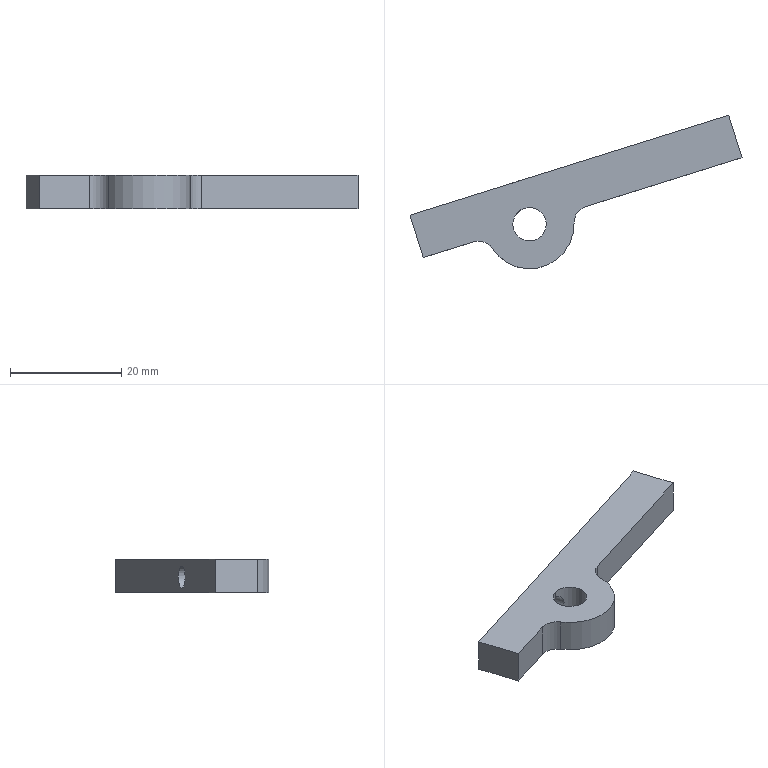Component | SolidWorks | Handle.1-1 | 1 solid | 16 faces | box 59.65 x 27.59 x 6 mm | volume 3263 mm3 | cylinder 7 | plane 7 | cone 2 | commonest cylinder face diameters 6 x4 4 x2 16 x1
build123d program:
from build123d import *

# Parameters (mm, degrees)
SKETCH1_R                   = 3
BOSS_EXTRUDE1_DEPTH         = 6
M4_TAPPED_HOLE1_D           = 3.3
M4_TAPPED_HOLE1_DEPTH       = 10.1
M4_TAPPED_HOLE1_CBORE_D     = 4
M4_TAPPED_HOLE1_CBORE_DEPTH = 8
M4_TAPPED_HOLE1_TIP         = 0.9914


with BuildPart() as part:
    # Sketch1 → Boss-Extrude1 (new body)
    with BuildSketch(Plane.XY):
        with BuildLine():
            Line((3, 24.417), (3, 15))
            Line((3, 15), (-5, 15))
            Line((-5, 15), (-5, 75))
            Line((-5, 75), (3, 75))
            Line((3, 75), (3, 45.583))
            ThreePointArc((3, 45.583), (3.607, 43.774), (5.182, 42.697))
            ThreePointArc((5.182, 42.697), (11, 35), (5.182, 27.303))
            ThreePointArc((5.182, 27.303), (3.607, 26.226), (3, 24.417))
        make_face()
        with Locations((3, 35)):
            Circle(SKETCH1_R, mode=Mode.SUBTRACT)
    extrude(amount=BOSS_EXTRUDE1_DEPTH)

    # M4 Tapped Hole1
    with Locations(Plane.ZY.offset(5)):
        with Locations((2.791, 35)):
            CounterBoreHole(M4_TAPPED_HOLE1_D / 2, M4_TAPPED_HOLE1_CBORE_D / 2, M4_TAPPED_HOLE1_CBORE_DEPTH, depth=M4_TAPPED_HOLE1_DEPTH)
            with Locations((0, 0, -(M4_TAPPED_HOLE1_DEPTH + M4_TAPPED_HOLE1_TIP / 2))):  # 118° drill point
                Cone(0, M4_TAPPED_HOLE1_D / 2, M4_TAPPED_HOLE1_TIP, mode=Mode.SUBTRACT)


solid = part.part

# Placed as in the assembly
solid = solid.moved(Location((30.703, 192.405, -88), (0, 0, -72.614)))
STEP:
#1=CARTESIAN_POINT('',(2.524,7.987,-3.276));
#2=VERTEX_POINT('',#1);
#3=CARTESIAN_POINT('',(2.524,7.987,-3.433));
#4=VERTEX_POINT('',#3);
#5=CARTESIAN_POINT('',(2.524,7.987,-3.276));
#6=CARTESIAN_POINT('',(2.519,7.985,-3.276));
#7=CARTESIAN_POINT('',(2.514,7.983,-3.277));
#8=CARTESIAN_POINT('',(2.504,7.979,-3.279));
#9=CARTESIAN_POINT('',(2.5,7.976,-3.28));
#10=CARTESIAN_POINT('',(2.487,7.968,-3.286));
#11=CARTESIAN_POINT('',(2.48,7.962,-3.292));
#12=CARTESIAN_POINT('',(2.472,7.954,-3.303));
#13=CARTESIAN_POINT('',(2.469,7.951,-3.307));
#14=CARTESIAN_POINT('',(2.465,7.946,-3.315));
#15=CARTESIAN_POINT('',(2.463,7.943,-3.319));
#16=CARTESIAN_POINT('',(2.461,7.939,-3.329));
#17=CARTESIAN_POINT('',(2.459,7.938,-3.334));
#18=CARTESIAN_POINT('',(2.458,7.935,-3.344));
#19=CARTESIAN_POINT('',(2.458,7.935,-3.349));
#20=CARTESIAN_POINT('',(2.458,7.934,-3.365));
#21=CARTESIAN_POINT('',(2.459,7.937,-3.376));
#22=CARTESIAN_POINT('',(2.465,7.945,-3.395));
#23=CARTESIAN_POINT('',(2.469,7.951,-3.403));
#24=CARTESIAN_POINT('',(2.477,7.96,-3.414));
#25=CARTESIAN_POINT('',(2.481,7.962,-3.417));
#26=CARTESIAN_POINT('',(2.488,7.968,-3.423));
#27=CARTESIAN_POINT('',(2.491,7.971,-3.425));
#28=CARTESIAN_POINT('',(2.5,7.976,-3.429));
#29=CARTESIAN_POINT('',(2.504,7.979,-3.431));
#30=CARTESIAN_POINT('',(2.514,7.983,-3.433));
#31=CARTESIAN_POINT('',(2.519,7.985,-3.433));
#32=CARTESIAN_POINT('',(2.524,7.987,-3.433));
#33=B_SPLINE_CURVE_WITH_KNOTS('',3,(#5,#6,#7,#8,#9,#10,#11,#12,#13,#14,#15,#16,#17,#18,#19,#20,#21,#22,#23,#24,#25,#26,#27,#28,#29,#30,#31,#32),.UNSPECIFIED.,.F.,.F.,(4,2,2,2,2,2,2,2,2,2,2,2,2,4),(0.,0.000404,0.000808,0.001616,0.00202,0.002424,0.002828,0.003232,0.00404,0.004848,0.005252,0.005656,0.00606,0.006464),.UNSPECIFIED.);
#34=EDGE_CURVE('',#2,#4,#33,.T.);
#35=ORIENTED_EDGE('',*,*,#34,.T.);
#36=CARTESIAN_POINT('',(2.465,8.175,-3.433));
#37=VERTEX_POINT('',#36);
#38=CARTESIAN_POINT('',(2.465,8.175,-3.433));
#39=DIRECTION('',(-0.2988,0.9543,0.));
#40=VECTOR('',#39,39.37);
#41=LINE('',#38,#40);
#42=EDGE_CURVE('',#4,#37,#41,.T.);
#43=ORIENTED_EDGE('',*,*,#42,.T.);
#44=CARTESIAN_POINT('',(2.465,8.175,-3.276));
#45=VERTEX_POINT('',#44);
#46=CARTESIAN_POINT('',(2.465,8.175,-3.355));
#47=DIRECTION('',(-0.2988,0.9543,0.));
#48=DIRECTION('',(0.,0.,1.));
#49=AXIS2_PLACEMENT_3D('',#46,#47,#48);
#50=CIRCLE('',#49,0.07874);
#51=EDGE_CURVE('',#37,#45,#50,.T.);
#52=ORIENTED_EDGE('',*,*,#51,.T.);
#53=CARTESIAN_POINT('',(2.465,8.175,-3.276));
#54=DIRECTION('',(-0.2988,0.9543,0.));
#55=VECTOR('',#54,39.37);
#56=LINE('',#53,#55);
#57=EDGE_CURVE('',#2,#45,#56,.T.);
#58=ORIENTED_EDGE('',*,*,#57,.F.);
#59=EDGE_LOOP('',(#35,#43,#52,#58));
#60=FACE_OUTER_BOUND('',#59,.T.);
#61=CARTESIAN_POINT('',(2.465,8.175,-3.355));
#62=DIRECTION('',(-0.2988,0.9543,0.));
#63=DIRECTION('',(0.,0.,1.));
#64=AXIS2_PLACEMENT_3D('',#61,#62,#63);
#65=CYLINDRICAL_SURFACE('',#64,0.07874);
#66=ADVANCED_FACE('',(#60),#65,.F.);
#67=CARTESIAN_POINT('',(2.595,7.758,-3.355));
#68=VERTEX_POINT('',#67);
#69=CARTESIAN_POINT('',(2.594,7.761,-3.349));
#70=VERTEX_POINT('',#69);
#71=CARTESIAN_POINT('',(2.584,7.795,-3.29));
#72=DIRECTION('',(-0.1539,0.4915,0.8572));
#73=VECTOR('',#72,39.37);
#74=LINE('',#71,#73);
#75=EDGE_CURVE('',#68,#70,#74,.T.);
#76=ORIENTED_EDGE('',*,*,#75,.F.);
#77=CARTESIAN_POINT('',(2.594,7.761,-3.361));
#78=VERTEX_POINT('',#77);
#79=CARTESIAN_POINT('',(2.584,7.795,-3.42));
#80=DIRECTION('',(-0.1539,0.4915,-0.8572));
#81=VECTOR('',#80,39.37);
#82=LINE('',#79,#81);
#83=EDGE_CURVE('',#68,#78,#82,.T.);
#84=ORIENTED_EDGE('',*,*,#83,.T.);
#85=CARTESIAN_POINT('',(2.594,7.761,-3.361));
#86=CARTESIAN_POINT('',(2.594,7.761,-3.361));
#87=CARTESIAN_POINT('',(2.593,7.761,-3.361));
#88=CARTESIAN_POINT('',(2.592,7.761,-3.36));
#89=CARTESIAN_POINT('',(2.592,7.76,-3.36));
#90=CARTESIAN_POINT('',(2.591,7.76,-3.36));
#91=CARTESIAN_POINT('',(2.59,7.76,-3.359));
#92=CARTESIAN_POINT('',(2.59,7.76,-3.359));
#93=CARTESIAN_POINT('',(2.59,7.76,-3.358));
#94=CARTESIAN_POINT('',(2.589,7.76,-3.358));
#95=CARTESIAN_POINT('',(2.589,7.76,-3.358));
#96=CARTESIAN_POINT('',(2.589,7.76,-3.357));
#97=CARTESIAN_POINT('',(2.589,7.76,-3.357));
#98=CARTESIAN_POINT('',(2.588,7.76,-3.356));
#99=CARTESIAN_POINT('',(2.588,7.76,-3.355));
#100=CARTESIAN_POINT('',(2.588,7.76,-3.355));
#101=CARTESIAN_POINT('',(2.588,7.76,-3.354));
#102=CARTESIAN_POINT('',(2.588,7.76,-3.353));
#103=CARTESIAN_POINT('',(2.589,7.76,-3.353));
#104=CARTESIAN_POINT('',(2.589,7.76,-3.352));
#105=CARTESIAN_POINT('',(2.589,7.76,-3.351));
#106=CARTESIAN_POINT('',(2.59,7.76,-3.351));
#107=CARTESIAN_POINT('',(2.59,7.76,-3.35));
#108=CARTESIAN_POINT('',(2.591,7.76,-3.35));
#109=CARTESIAN_POINT('',(2.591,7.76,-3.35));
#110=CARTESIAN_POINT('',(2.592,7.76,-3.349));
#111=CARTESIAN_POINT('',(2.592,7.761,-3.349));
#112=CARTESIAN_POINT('',(2.593,7.761,-3.349));
#113=CARTESIAN_POINT('',(2.593,7.761,-3.349));
#114=CARTESIAN_POINT('',(2.594,7.761,-3.349));
#115=CARTESIAN_POINT('',(2.594,7.761,-3.349));
#116=B_SPLINE_CURVE_WITH_KNOTS('',3,(#85,#86,#87,#88,#89,#90,#91,#92,#93,#94,#95,#96,#97,#98,#99,#100,#101,#102,#103,#104,#105,#106,#107,#108,#109,#110,#111,#112,#113,#114,#115),.UNSPECIFIED.,.F.,.F.,(4,3,3,3,3,3,3,3,3,3,4),(0.0008224,0.0008771,0.0009329,0.0009775,0.00102,0.001071,0.00112,0.001169,0.001219,0.001272,0.001311),.UNSPECIFIED.);
#117=EDGE_CURVE('',#78,#70,#116,.T.);
#118=ORIENTED_EDGE('',*,*,#117,.T.);
#119=EDGE_LOOP('',(#76,#84,#118));
#120=FACE_OUTER_BOUND('',#119,.T.);
#121=CARTESIAN_POINT('',(2.584,7.795,-3.355));
#122=DIRECTION('',(-0.2988,0.9543,0.));
#123=DIRECTION('',(0.,0.,1.));
#124=AXIS2_PLACEMENT_3D('',#121,#122,#123);
#125=CONICAL_SURFACE('',#124,0.06496,1.03);
#126=ADVANCED_FACE('',(#120),#125,.F.);
#127=CARTESIAN_POINT('',(2.524,7.987,-3.228));
#128=VERTEX_POINT('',#127);
#129=CARTESIAN_POINT('',(2.594,7.761,-3.228));
#130=VERTEX_POINT('',#129);
#131=CARTESIAN_POINT('',(2.559,7.874,-3.228));
#132=DIRECTION('',(0.,-0.,1.));
#133=DIRECTION('',(0.2988,-0.9543,0.));
#134=AXIS2_PLACEMENT_3D('',#131,#132,#133);
#135=CIRCLE('',#134,0.1181);
#136=EDGE_CURVE('',#128,#130,#135,.T.);
#137=ORIENTED_EDGE('',*,*,#136,.T.);
#138=CARTESIAN_POINT('',(2.594,7.761,-3.228));
#139=DIRECTION('',(-0.,0.,-1.));
#140=VECTOR('',#139,39.37);
#141=LINE('',#138,#140);
#142=EDGE_CURVE('',#130,#70,#141,.T.);
#143=ORIENTED_EDGE('',*,*,#142,.T.);
#144=ORIENTED_EDGE('',*,*,#117,.F.);
#145=CARTESIAN_POINT('',(2.594,7.761,-3.465));
#146=VERTEX_POINT('',#145);
#147=CARTESIAN_POINT('',(2.594,7.761,-3.228));
#148=DIRECTION('',(-0.,0.,-1.));
#149=VECTOR('',#148,39.37);
#150=LINE('',#147,#149);
#151=EDGE_CURVE('',#78,#146,#150,.T.);
#152=ORIENTED_EDGE('',*,*,#151,.T.);
#153=CARTESIAN_POINT('',(2.524,7.987,-3.465));
#154=VERTEX_POINT('',#153);
#155=CARTESIAN_POINT('',(2.559,7.874,-3.465));
#156=DIRECTION('',(0.,-0.,1.));
#157=DIRECTION('',(0.2988,-0.9543,0.));
#158=AXIS2_PLACEMENT_3D('',#155,#156,#157);
#159=CIRCLE('',#158,0.1181);
#160=EDGE_CURVE('',#154,#146,#159,.T.);
#161=ORIENTED_EDGE('',*,*,#160,.F.);
#162=CARTESIAN_POINT('',(2.524,7.987,-3.228));
#163=DIRECTION('',(-0.,0.,-1.));
#164=VECTOR('',#163,39.37);
#165=LINE('',#162,#164);
#166=EDGE_CURVE('',#4,#154,#165,.T.);
#167=ORIENTED_EDGE('',*,*,#166,.F.);
#168=ORIENTED_EDGE('',*,*,#34,.F.);
#169=CARTESIAN_POINT('',(2.524,7.987,-3.228));
#170=DIRECTION('',(-0.,0.,-1.));
#171=VECTOR('',#170,39.37);
#172=LINE('',#169,#171);
#173=EDGE_CURVE('',#128,#2,#172,.T.);
#174=ORIENTED_EDGE('',*,*,#173,.F.);
#175=EDGE_LOOP('',(#137,#143,#144,#152,#161,#167,#168,#174));
#176=FACE_OUTER_BOUND('',#175,.T.);
#177=CARTESIAN_POINT('',(2.559,7.874,-3.228));
#178=DIRECTION('',(-0.,0.,-1.));
#179=DIRECTION('',(-0.2988,0.9543,0.));
#180=AXIS2_PLACEMENT_3D('',#177,#178,#179);
#181=CYLINDRICAL_SURFACE('',#180,0.1181);
#182=ADVANCED_FACE('',(#176),#181,.F.);
#183=CARTESIAN_POINT('',(1.714,7.939,-3.228));
#184=VERTEX_POINT('',#183);
#185=CARTESIAN_POINT('',(1.808,7.639,-3.228));
#186=VERTEX_POINT('',#185);
#187=CARTESIAN_POINT('',(1.714,7.939,-3.228));
#188=DIRECTION('',(0.2988,-0.9543,-0.));
#189=VECTOR('',#188,39.37);
#190=LINE('',#187,#189);
#191=EDGE_CURVE('',#184,#186,#190,.T.);
#192=ORIENTED_EDGE('',*,*,#191,.T.);
#193=CARTESIAN_POINT('',(2.161,7.75,-3.228));
#194=VERTEX_POINT('',#193);
#195=CARTESIAN_POINT('',(2.161,7.75,-3.228));
#196=DIRECTION('',(0.9543,0.2988,-0.));
#197=VECTOR('',#196,39.37);
#198=LINE('',#195,#197);
#199=EDGE_CURVE('',#186,#194,#198,.T.);
#200=ORIENTED_EDGE('',*,*,#199,.T.);
#201=CARTESIAN_POINT('',(2.296,7.701,-3.228));
#202=VERTEX_POINT('',#201);
#203=CARTESIAN_POINT('',(2.197,7.637,-3.228));
#204=DIRECTION('',(-0.,0.,-1.));
#205=DIRECTION('',(0.2988,-0.9543,0.));
#206=AXIS2_PLACEMENT_3D('',#203,#204,#205);
#207=CIRCLE('',#206,0.1181);
#208=EDGE_CURVE('',#194,#202,#207,.T.);
#209=ORIENTED_EDGE('',*,*,#208,.T.);
#210=CARTESIAN_POINT('',(2.874,7.883,-3.228));
#211=VERTEX_POINT('',#210);
#212=CARTESIAN_POINT('',(2.559,7.874,-3.228));
#213=DIRECTION('',(0.,-0.,1.));
#214=DIRECTION('',(0.2988,-0.9543,0.));
#215=AXIS2_PLACEMENT_3D('',#212,#213,#214);
#216=CIRCLE('',#215,0.315);
#217=EDGE_CURVE('',#202,#211,#216,.T.);
#218=ORIENTED_EDGE('',*,*,#217,.T.);
#219=CARTESIAN_POINT('',(2.957,7.999,-3.228));
#220=VERTEX_POINT('',#219);
#221=CARTESIAN_POINT('',(2.992,7.886,-3.228));
#222=DIRECTION('',(-0.,0.,-1.));
#223=DIRECTION('',(0.2988,-0.9543,0.));
#224=AXIS2_PLACEMENT_3D('',#221,#222,#223);
#225=CIRCLE('',#224,0.1181);
#226=EDGE_CURVE('',#211,#220,#225,.T.);
#227=ORIENTED_EDGE('',*,*,#226,.T.);
#228=CARTESIAN_POINT('',(4.062,8.345,-3.228));
#229=VERTEX_POINT('',#228);
#230=CARTESIAN_POINT('',(4.062,8.345,-3.228));
#231=DIRECTION('',(0.9543,0.2988,-0.));
#232=VECTOR('',#231,39.37);
#233=LINE('',#230,#232);
#234=EDGE_CURVE('',#220,#229,#233,.T.);
#235=ORIENTED_EDGE('',*,*,#234,.T.);
#236=CARTESIAN_POINT('',(3.968,8.645,-3.228));
#237=VERTEX_POINT('',#236);
#238=CARTESIAN_POINT('',(3.968,8.645,-3.228));
#239=DIRECTION('',(-0.2988,0.9543,0.));
#240=VECTOR('',#239,39.37);
#241=LINE('',#238,#240);
#242=EDGE_CURVE('',#229,#237,#241,.T.);
#243=ORIENTED_EDGE('',*,*,#242,.T.);
#244=CARTESIAN_POINT('',(3.968,8.645,-3.228));
#245=DIRECTION('',(-0.9543,-0.2988,0.));
#246=VECTOR('',#245,39.37);
#247=LINE('',#244,#246);
#248=EDGE_CURVE('',#237,#184,#247,.T.);
#249=ORIENTED_EDGE('',*,*,#248,.T.);
#250=EDGE_LOOP('',(#192,#200,#209,#218,#227,#235,#243,#249));
#251=FACE_OUTER_BOUND('',#250,.T.);
#252=ORIENTED_EDGE('',*,*,#136,.F.);
#253=CARTESIAN_POINT('',(2.559,7.874,-3.228));
#254=DIRECTION('',(0.,-0.,1.));
#255=DIRECTION('',(0.2988,-0.9543,0.));
#256=AXIS2_PLACEMENT_3D('',#253,#254,#255);
#257=CIRCLE('',#256,0.1181);
#258=EDGE_CURVE('',#130,#128,#257,.T.);
#259=ORIENTED_EDGE('',*,*,#258,.F.);
#260=EDGE_LOOP('',(#252,#259));
#261=FACE_BOUND('',#260,.T.);
#262=CARTESIAN_POINT('',(2.197,7.637,-3.228));
#263=DIRECTION('',(0.,-0.,1.));
#264=DIRECTION('',(0.2988,-0.9543,-0.));
#265=AXIS2_PLACEMENT_3D('',#262,#263,#264);
#266=PLANE('',#265);
#267=ADVANCED_FACE('',(#251,#261),#266,.T.);
#268=CARTESIAN_POINT('',(1.714,7.939,-3.465));
#269=VERTEX_POINT('',#268);
#270=CARTESIAN_POINT('',(1.808,7.639,-3.465));
#271=VERTEX_POINT('',#270);
#272=CARTESIAN_POINT('',(1.714,7.939,-3.465));
#273=DIRECTION('',(0.2988,-0.9543,-0.));
#274=VECTOR('',#273,39.37);
#275=LINE('',#272,#274);
#276=EDGE_CURVE('',#269,#271,#275,.T.);
#277=ORIENTED_EDGE('',*,*,#276,.F.);
#278=CARTESIAN_POINT('',(3.968,8.645,-3.465));
#279=VERTEX_POINT('',#278);
#280=CARTESIAN_POINT('',(3.968,8.645,-3.465));
#281=DIRECTION('',(-0.9543,-0.2988,0.));
#282=VECTOR('',#281,39.37);
#283=LINE('',#280,#282);
#284=EDGE_CURVE('',#279,#269,#283,.T.);
#285=ORIENTED_EDGE('',*,*,#284,.F.);
#286=CARTESIAN_POINT('',(4.062,8.345,-3.465));
#287=VERTEX_POINT('',#286);
#288=CARTESIAN_POINT('',(3.968,8.645,-3.465));
#289=DIRECTION('',(-0.2988,0.9543,0.));
#290=VECTOR('',#289,39.37);
#291=LINE('',#288,#290);
#292=EDGE_CURVE('',#287,#279,#291,.T.);
#293=ORIENTED_EDGE('',*,*,#292,.F.);
#294=CARTESIAN_POINT('',(2.957,7.999,-3.465));
#295=VERTEX_POINT('',#294);
#296=CARTESIAN_POINT('',(4.062,8.345,-3.465));
#297=DIRECTION('',(0.9543,0.2988,-0.));
#298=VECTOR('',#297,39.37);
#299=LINE('',#296,#298);
#300=EDGE_CURVE('',#295,#287,#299,.T.);
#301=ORIENTED_EDGE('',*,*,#300,.F.);
#302=CARTESIAN_POINT('',(2.874,7.883,-3.465));
#303=VERTEX_POINT('',#302);
#304=CARTESIAN_POINT('',(2.992,7.886,-3.465));
#305=DIRECTION('',(-0.,0.,-1.));
#306=DIRECTION('',(0.2988,-0.9543,0.));
#307=AXIS2_PLACEMENT_3D('',#304,#305,#306);
#308=CIRCLE('',#307,0.1181);
#309=EDGE_CURVE('',#303,#295,#308,.T.);
#310=ORIENTED_EDGE('',*,*,#309,.F.);
#311=CARTESIAN_POINT('',(2.296,7.701,-3.465));
#312=VERTEX_POINT('',#311);
#313=CARTESIAN_POINT('',(2.559,7.874,-3.465));
#314=DIRECTION('',(0.,-0.,1.));
#315=DIRECTION('',(0.2988,-0.9543,0.));
#316=AXIS2_PLACEMENT_3D('',#313,#314,#315);
#317=CIRCLE('',#316,0.315);
#318=EDGE_CURVE('',#312,#303,#317,.T.);
#319=ORIENTED_EDGE('',*,*,#318,.F.);
#320=CARTESIAN_POINT('',(2.161,7.75,-3.465));
#321=VERTEX_POINT('',#320);
#322=CARTESIAN_POINT('',(2.197,7.637,-3.465));
#323=DIRECTION('',(-0.,0.,-1.));
#324=DIRECTION('',(0.2988,-0.9543,0.));
#325=AXIS2_PLACEMENT_3D('',#322,#323,#324);
#326=CIRCLE('',#325,0.1181);
#327=EDGE_CURVE('',#321,#312,#326,.T.);
#328=ORIENTED_EDGE('',*,*,#327,.F.);
#329=CARTESIAN_POINT('',(2.161,7.75,-3.465));
#330=DIRECTION('',(0.9543,0.2988,-0.));
#331=VECTOR('',#330,39.37);
#332=LINE('',#329,#331);
#333=EDGE_CURVE('',#271,#321,#332,.T.);
#334=ORIENTED_EDGE('',*,*,#333,.F.);
#335=EDGE_LOOP('',(#277,#285,#293,#301,#310,#319,#328,#334));
#336=FACE_OUTER_BOUND('',#335,.T.);
#337=ORIENTED_EDGE('',*,*,#160,.T.);
#338=CARTESIAN_POINT('',(2.559,7.874,-3.465));
#339=DIRECTION('',(0.,-0.,1.));
#340=DIRECTION('',(0.2988,-0.9543,0.));
#341=AXIS2_PLACEMENT_3D('',#338,#339,#340);
#342=CIRCLE('',#341,0.1181);
#343=EDGE_CURVE('',#146,#154,#342,.T.);
#344=ORIENTED_EDGE('',*,*,#343,.T.);
#345=EDGE_LOOP('',(#337,#344));
#346=FACE_BOUND('',#345,.T.);
#347=CARTESIAN_POINT('',(2.197,7.637,-3.465));
#348=DIRECTION('',(0.,-0.,1.));
#349=DIRECTION('',(0.2988,-0.9543,-0.));
#350=AXIS2_PLACEMENT_3D('',#347,#348,#349);
#351=PLANE('',#350);
#352=ADVANCED_FACE('',(#336,#346),#351,.F.);
#353=ORIENTED_EDGE('',*,*,#276,.T.);
#354=CARTESIAN_POINT('',(1.808,7.639,-3.228));
#355=DIRECTION('',(-0.,0.,-1.));
#356=VECTOR('',#355,39.37);
#357=LINE('',#354,#356);
#358=EDGE_CURVE('',#186,#271,#357,.T.);
#359=ORIENTED_EDGE('',*,*,#358,.F.);
#360=ORIENTED_EDGE('',*,*,#191,.F.);
#361=CARTESIAN_POINT('',(1.714,7.939,-3.228));
#362=DIRECTION('',(-0.,0.,-1.));
#363=VECTOR('',#362,39.37);
#364=LINE('',#361,#363);
#365=EDGE_CURVE('',#184,#269,#364,.T.);
#366=ORIENTED_EDGE('',*,*,#365,.T.);
#367=EDGE_LOOP('',(#353,#359,#360,#366));
#368=FACE_OUTER_BOUND('',#367,.T.);
#369=CARTESIAN_POINT('',(1.714,7.939,-3.228));
#370=DIRECTION('',(0.9543,0.2988,-0.));
#371=DIRECTION('',(0.,-0.,1.));
#372=AXIS2_PLACEMENT_3D('',#369,#370,#371);
#373=PLANE('',#372);
#374=ADVANCED_FACE('',(#368),#373,.F.);
#375=ORIENTED_EDGE('',*,*,#333,.T.);
#376=CARTESIAN_POINT('',(2.161,7.75,-3.228));
#377=DIRECTION('',(-0.,0.,-1.));
#378=VECTOR('',#377,39.37);
#379=LINE('',#376,#378);
#380=EDGE_CURVE('',#194,#321,#379,.T.);
#381=ORIENTED_EDGE('',*,*,#380,.F.);
#382=ORIENTED_EDGE('',*,*,#199,.F.);
#383=ORIENTED_EDGE('',*,*,#358,.T.);
#384=EDGE_LOOP('',(#375,#381,#382,#383));
#385=FACE_OUTER_BOUND('',#384,.T.);
#386=CARTESIAN_POINT('',(2.161,7.75,-3.228));
#387=DIRECTION('',(-0.2988,0.9543,0.));
#388=DIRECTION('',(-0.9543,-0.2988,0.));
#389=AXIS2_PLACEMENT_3D('',#386,#387,#388);
#390=PLANE('',#389);
#391=ADVANCED_FACE('',(#385),#390,.F.);
#392=ORIENTED_EDGE('',*,*,#327,.T.);
#393=CARTESIAN_POINT('',(2.296,7.701,-3.228));
#394=DIRECTION('',(-0.,0.,-1.));
#395=VECTOR('',#394,39.37);
#396=LINE('',#393,#395);
#397=EDGE_CURVE('',#202,#312,#396,.T.);
#398=ORIENTED_EDGE('',*,*,#397,.F.);
#399=ORIENTED_EDGE('',*,*,#208,.F.);
#400=ORIENTED_EDGE('',*,*,#380,.T.);
#401=EDGE_LOOP('',(#392,#398,#399,#400));
#402=FACE_OUTER_BOUND('',#401,.T.);
#403=CARTESIAN_POINT('',(2.197,7.637,-3.228));
#404=DIRECTION('',(-0.,0.,-1.));
#405=DIRECTION('',(-0.2988,0.9543,0.));
#406=AXIS2_PLACEMENT_3D('',#403,#404,#405);
#407=CYLINDRICAL_SURFACE('',#406,0.1181);
#408=ADVANCED_FACE('',(#402),#407,.F.);
#409=ORIENTED_EDGE('',*,*,#318,.T.);
#410=CARTESIAN_POINT('',(2.874,7.883,-3.228));
#411=DIRECTION('',(-0.,0.,-1.));
#412=VECTOR('',#411,39.37);
#413=LINE('',#410,#412);
#414=EDGE_CURVE('',#211,#303,#413,.T.);
#415=ORIENTED_EDGE('',*,*,#414,.F.);
#416=ORIENTED_EDGE('',*,*,#217,.F.);
#417=ORIENTED_EDGE('',*,*,#397,.T.);
#418=EDGE_LOOP('',(#409,#415,#416,#417));
#419=FACE_OUTER_BOUND('',#418,.T.);
#420=CARTESIAN_POINT('',(2.559,7.874,-3.228));
#421=DIRECTION('',(-0.,0.,-1.));
#422=DIRECTION('',(-0.2988,0.9543,0.));
#423=AXIS2_PLACEMENT_3D('',#420,#421,#422);
#424=CYLINDRICAL_SURFACE('',#423,0.315);
#425=ADVANCED_FACE('',(#419),#424,.T.);
#426=ORIENTED_EDGE('',*,*,#309,.T.);
#427=CARTESIAN_POINT('',(2.957,7.999,-3.228));
#428=DIRECTION('',(-0.,0.,-1.));
#429=VECTOR('',#428,39.37);
#430=LINE('',#427,#429);
#431=EDGE_CURVE('',#220,#295,#430,.T.);
#432=ORIENTED_EDGE('',*,*,#431,.F.);
#433=ORIENTED_EDGE('',*,*,#226,.F.);
#434=ORIENTED_EDGE('',*,*,#414,.T.);
#435=EDGE_LOOP('',(#426,#432,#433,#434));
#436=FACE_OUTER_BOUND('',#435,.T.);
#437=CARTESIAN_POINT('',(2.992,7.886,-3.228));
#438=DIRECTION('',(-0.,0.,-1.));
#439=DIRECTION('',(-0.2988,0.9543,0.));
#440=AXIS2_PLACEMENT_3D('',#437,#438,#439);
#441=CYLINDRICAL_SURFACE('',#440,0.1181);
#442=ADVANCED_FACE('',(#436),#441,.F.);
#443=ORIENTED_EDGE('',*,*,#300,.T.);
#444=CARTESIAN_POINT('',(4.062,8.345,-3.228));
#445=DIRECTION('',(-0.,0.,-1.));
#446=VECTOR('',#445,39.37);
#447=LINE('',#444,#446);
#448=EDGE_CURVE('',#229,#287,#447,.T.);
#449=ORIENTED_EDGE('',*,*,#448,.F.);
#450=ORIENTED_EDGE('',*,*,#234,.F.);
#451=ORIENTED_EDGE('',*,*,#431,.T.);
#452=EDGE_LOOP('',(#443,#449,#450,#451));
#453=FACE_OUTER_BOUND('',#452,.T.);
#454=CARTESIAN_POINT('',(4.062,8.345,-3.228));
#455=DIRECTION('',(-0.2988,0.9543,0.));
#456=DIRECTION('',(-0.9543,-0.2988,0.));
#457=AXIS2_PLACEMENT_3D('',#454,#455,#456);
#458=PLANE('',#457);
#459=ADVANCED_FACE('',(#453),#458,.F.);
#460=ORIENTED_EDGE('',*,*,#292,.T.);
#461=CARTESIAN_POINT('',(3.968,8.645,-3.228));
#462=DIRECTION('',(-0.,0.,-1.));
#463=VECTOR('',#462,39.37);
#464=LINE('',#461,#463);
#465=EDGE_CURVE('',#237,#279,#464,.T.);
#466=ORIENTED_EDGE('',*,*,#465,.F.);
#467=ORIENTED_EDGE('',*,*,#242,.F.);
#468=ORIENTED_EDGE('',*,*,#448,.T.);
#469=EDGE_LOOP('',(#460,#466,#467,#468));
#470=FACE_OUTER_BOUND('',#469,.T.);
#471=CARTESIAN_POINT('',(3.968,8.645,-3.228));
#472=DIRECTION('',(-0.9543,-0.2988,0.));
#473=DIRECTION('',(-0.,0.,-1.));
#474=AXIS2_PLACEMENT_3D('',#471,#472,#473);
#475=PLANE('',#474);
#476=ADVANCED_FACE('',(#470),#475,.F.);
#477=CARTESIAN_POINT('',(2.465,8.175,-3.355));
#478=DIRECTION('',(-0.2988,0.9543,0.));
#479=DIRECTION('',(0.,0.,1.));
#480=AXIS2_PLACEMENT_3D('',#477,#478,#479);
#481=CIRCLE('',#480,0.07874);
#482=EDGE_CURVE('',#45,#37,#481,.T.);
#483=ORIENTED_EDGE('',*,*,#482,.F.);
#484=ORIENTED_EDGE('',*,*,#51,.F.);
#485=EDGE_LOOP('',(#483,#484));
#486=FACE_BOUND('',#485,.T.);
#487=ORIENTED_EDGE('',*,*,#284,.T.);
#488=ORIENTED_EDGE('',*,*,#365,.F.);
#489=ORIENTED_EDGE('',*,*,#248,.F.);
#490=ORIENTED_EDGE('',*,*,#465,.T.);
#491=EDGE_LOOP('',(#487,#488,#489,#490));
#492=FACE_OUTER_BOUND('',#491,.T.);
#493=CARTESIAN_POINT('',(3.968,8.645,-3.228));
#494=DIRECTION('',(0.2988,-0.9543,-0.));
#495=DIRECTION('',(0.9543,0.2988,-0.));
#496=AXIS2_PLACEMENT_3D('',#493,#494,#495);
#497=PLANE('',#496);
#498=ADVANCED_FACE('',(#486,#492),#497,.F.);
#499=ORIENTED_EDGE('',*,*,#142,.F.);
#500=ORIENTED_EDGE('',*,*,#258,.T.);
#501=ORIENTED_EDGE('',*,*,#173,.T.);
#502=CARTESIAN_POINT('',(2.524,7.987,-3.433));
#503=CARTESIAN_POINT('',(2.529,7.988,-3.433));
#504=CARTESIAN_POINT('',(2.534,7.99,-3.433));
#505=CARTESIAN_POINT('',(2.544,7.991,-3.431));
#506=CARTESIAN_POINT('',(2.549,7.992,-3.429));
#507=CARTESIAN_POINT('',(2.564,7.992,-3.423));
#508=CARTESIAN_POINT('',(2.573,7.992,-3.417));
#509=CARTESIAN_POINT('',(2.585,7.989,-3.407));
#510=CARTESIAN_POINT('',(2.589,7.988,-3.403));
#511=CARTESIAN_POINT('',(2.595,7.986,-3.394));
#512=CARTESIAN_POINT('',(2.598,7.986,-3.39));
#513=CARTESIAN_POINT('',(2.603,7.984,-3.381));
#514=CARTESIAN_POINT('',(2.605,7.983,-3.376));
#515=CARTESIAN_POINT('',(2.607,7.982,-3.365));
#516=CARTESIAN_POINT('',(2.608,7.982,-3.36));
#517=CARTESIAN_POINT('',(2.608,7.982,-3.349));
#518=CARTESIAN_POINT('',(2.607,7.982,-3.344));
#519=CARTESIAN_POINT('',(2.605,7.983,-3.334));
#520=CARTESIAN_POINT('',(2.603,7.984,-3.329));
#521=CARTESIAN_POINT('',(2.596,7.986,-3.315));
#522=CARTESIAN_POINT('',(2.589,7.989,-3.306));
#523=CARTESIAN_POINT('',(2.577,7.991,-3.296));
#524=CARTESIAN_POINT('',(2.573,7.991,-3.292));
#525=CARTESIAN_POINT('',(2.564,7.992,-3.287));
#526=CARTESIAN_POINT('',(2.559,7.992,-3.284));
#527=CARTESIAN_POINT('',(2.55,7.992,-3.28));
#528=CARTESIAN_POINT('',(2.544,7.991,-3.279));
#529=CARTESIAN_POINT('',(2.534,7.99,-3.277));
#530=CARTESIAN_POINT('',(2.529,7.988,-3.276));
#531=CARTESIAN_POINT('',(2.524,7.987,-3.276));
#532=B_SPLINE_CURVE_WITH_KNOTS('',3,(#502,#503,#504,#505,#506,#507,#508,#509,#510,#511,#512,#513,#514,#515,#516,#517,#518,#519,#520,#521,#522,#523,#524,#525,#526,#527,#528,#529,#530,#531),.UNSPECIFIED.,.F.,.F.,(4,2,2,2,2,2,2,2,2,2,2,2,2,2,4),(0.006464,0.006867,0.007271,0.008078,0.008481,0.008885,0.009288,0.009692,0.0101,0.0105,0.01131,0.01171,0.01211,0.01252,0.01292),.UNSPECIFIED.);
#533=EDGE_CURVE('',#4,#2,#532,.T.);
#534=ORIENTED_EDGE('',*,*,#533,.F.);
#535=ORIENTED_EDGE('',*,*,#166,.T.);
#536=ORIENTED_EDGE('',*,*,#343,.F.);
#537=ORIENTED_EDGE('',*,*,#151,.F.);
#538=CARTESIAN_POINT('',(2.594,7.761,-3.349));
#539=CARTESIAN_POINT('',(2.595,7.761,-3.349));
#540=CARTESIAN_POINT('',(2.595,7.761,-3.349));
#541=CARTESIAN_POINT('',(2.595,7.761,-3.349));
#542=CARTESIAN_POINT('',(2.596,7.762,-3.349));
#543=CARTESIAN_POINT('',(2.596,7.762,-3.349));
#544=CARTESIAN_POINT('',(2.597,7.762,-3.349));
#545=CARTESIAN_POINT('',(2.598,7.762,-3.35));
#546=CARTESIAN_POINT('',(2.598,7.763,-3.35));
#547=CARTESIAN_POINT('',(2.599,7.763,-3.351));
#548=CARTESIAN_POINT('',(2.599,7.763,-3.351));
#549=CARTESIAN_POINT('',(2.6,7.763,-3.352));
#550=CARTESIAN_POINT('',(2.6,7.763,-3.352));
#551=CARTESIAN_POINT('',(2.6,7.763,-3.353));
#552=CARTESIAN_POINT('',(2.6,7.763,-3.354));
#553=CARTESIAN_POINT('',(2.6,7.763,-3.354));
#554=CARTESIAN_POINT('',(2.6,7.763,-3.355));
#555=CARTESIAN_POINT('',(2.6,7.763,-3.356));
#556=CARTESIAN_POINT('',(2.6,7.763,-3.356));
#557=CARTESIAN_POINT('',(2.6,7.763,-3.357));
#558=CARTESIAN_POINT('',(2.6,7.763,-3.357));
#559=CARTESIAN_POINT('',(2.599,7.763,-3.358));
#560=CARTESIAN_POINT('',(2.599,7.763,-3.358));
#561=CARTESIAN_POINT('',(2.599,7.763,-3.359));
#562=CARTESIAN_POINT('',(2.598,7.763,-3.359));
#563=CARTESIAN_POINT('',(2.598,7.762,-3.36));
#564=CARTESIAN_POINT('',(2.597,7.762,-3.36));
#565=CARTESIAN_POINT('',(2.596,7.762,-3.36));
#566=CARTESIAN_POINT('',(2.596,7.762,-3.361));
#567=CARTESIAN_POINT('',(2.595,7.762,-3.361));
#568=CARTESIAN_POINT('',(2.594,7.761,-3.361));
#569=CARTESIAN_POINT('',(2.594,7.761,-3.361));
#570=CARTESIAN_POINT('',(2.594,7.761,-3.361));
#571=CARTESIAN_POINT('',(2.594,7.761,-3.361));
#572=B_SPLINE_CURVE_WITH_KNOTS('',3,(#538,#539,#540,#541,#542,#543,#544,#545,#546,#547,#548,#549,#550,#551,#552,#553,#554,#555,#556,#557,#558,#559,#560,#561,#562,#563,#564,#565,#566,#567,#568,#569,#570,#571),.UNSPECIFIED.,.F.,.F.,(4,3,3,3,3,3,3,3,3,3,3,4),(0.0003336,0.0003498,0.0004057,0.0004613,0.0005151,0.0005665,0.0006159,0.0006648,0.0007149,0.000767,0.0008214,0.0008224),.UNSPECIFIED.);
#573=EDGE_CURVE('',#70,#78,#572,.T.);
#574=ORIENTED_EDGE('',*,*,#573,.F.);
#575=EDGE_LOOP('',(#499,#500,#501,#534,#535,#536,#537,#574));
#576=FACE_OUTER_BOUND('',#575,.T.);
#577=CARTESIAN_POINT('',(2.559,7.874,-3.228));
#578=DIRECTION('',(-0.,0.,-1.));
#579=DIRECTION('',(-0.2988,0.9543,0.));
#580=AXIS2_PLACEMENT_3D('',#577,#578,#579);
#581=CYLINDRICAL_SURFACE('',#580,0.1181);
#582=ADVANCED_FACE('',(#576),#581,.F.);
#583=ORIENTED_EDGE('',*,*,#83,.F.);
#584=ORIENTED_EDGE('',*,*,#75,.T.);
#585=ORIENTED_EDGE('',*,*,#573,.T.);
#586=EDGE_LOOP('',(#583,#584,#585));
#587=FACE_OUTER_BOUND('',#586,.T.);
#588=CARTESIAN_POINT('',(2.584,7.795,-3.355));
#589=DIRECTION('',(-0.2988,0.9543,0.));
#590=DIRECTION('',(0.,0.,1.));
#591=AXIS2_PLACEMENT_3D('',#588,#589,#590);
#592=CONICAL_SURFACE('',#591,0.06496,1.03);
#593=ADVANCED_FACE('',(#587),#592,.F.);
#594=ORIENTED_EDGE('',*,*,#42,.F.);
#595=ORIENTED_EDGE('',*,*,#533,.T.);
#596=ORIENTED_EDGE('',*,*,#57,.T.);
#597=ORIENTED_EDGE('',*,*,#482,.T.);
#598=EDGE_LOOP('',(#594,#595,#596,#597));
#599=FACE_OUTER_BOUND('',#598,.T.);
#600=CARTESIAN_POINT('',(2.465,8.175,-3.355));
#601=DIRECTION('',(-0.2988,0.9543,0.));
#602=DIRECTION('',(0.,0.,1.));
#603=AXIS2_PLACEMENT_3D('',#600,#601,#602);
#604=CYLINDRICAL_SURFACE('',#603,0.07874);
#605=ADVANCED_FACE('',(#599),#604,.F.);
#606=CLOSED_SHELL('',(#66,#126,#182,#267,#352,#374,#391,#408,#425,#442,#459,#476,#498,#582,#593,#605));
#607=MANIFOLD_SOLID_BREP('',#606);
#608=CARTESIAN_POINT('',(0.,0.,0.));
#609=DIRECTION('',(0.,0.,1.));
#610=DIRECTION('',(1.,0.,0.));
#611=AXIS2_PLACEMENT_3D('',#608,#609,#610);
#612=(LENGTH_UNIT()NAMED_UNIT(*)SI_UNIT($,.METRE.));
#613=LENGTH_MEASURE_WITH_UNIT(LENGTH_MEASURE(0.0254),#612);
#614=DIMENSIONAL_EXPONENTS(1.,0.,0.,0.,0.,0.,0.);
#615=(CONVERSION_BASED_UNIT('',#613)LENGTH_UNIT()NAMED_UNIT(#614));
#616=UNCERTAINTY_MEASURE_WITH_UNIT(LENGTH_MEASURE(0.00001),#615,'','');
#617=(NAMED_UNIT(*)PLANE_ANGLE_UNIT()SI_UNIT($,.RADIAN.));
#618=(NAMED_UNIT(*)SI_UNIT($,.STERADIAN.)SOLID_ANGLE_UNIT());
#619=(GEOMETRIC_REPRESENTATION_CONTEXT(3)GLOBAL_UNCERTAINTY_ASSIGNED_CONTEXT((#616))GLOBAL_UNIT_ASSIGNED_CONTEXT((#615,#617,#618))REPRESENTATION_CONTEXT('',''));
#620=ADVANCED_BREP_SHAPE_REPRESENTATION('',(#607,#611),#619);
#621=COLOUR_RGB('',0.7922,0.8196,0.9333);
#622=FILL_AREA_STYLE_COLOUR('',#621);
#623=FILL_AREA_STYLE('',(#622));
#624=SURFACE_STYLE_FILL_AREA(#623);
#625=SURFACE_SIDE_STYLE('',(#624));
#626=SURFACE_STYLE_USAGE(.BOTH.,#625);
#627=PRESENTATION_STYLE_ASSIGNMENT((#626));
#628=STYLED_ITEM('',(#627),#607);
#629=(LENGTH_UNIT()NAMED_UNIT(*)SI_UNIT($,.METRE.));
#630=LENGTH_MEASURE_WITH_UNIT(LENGTH_MEASURE(0.0254),#629);
#631=DIMENSIONAL_EXPONENTS(1.,0.,0.,0.,0.,0.,0.);
#632=(CONVERSION_BASED_UNIT('',#630)LENGTH_UNIT()NAMED_UNIT(#631));
#633=UNCERTAINTY_MEASURE_WITH_UNIT(LENGTH_MEASURE(0.00001),#632,'','');
#634=(NAMED_UNIT(*)PLANE_ANGLE_UNIT()SI_UNIT($,.RADIAN.));
#635=(NAMED_UNIT(*)SI_UNIT($,.STERADIAN.)SOLID_ANGLE_UNIT());
#636=(GEOMETRIC_REPRESENTATION_CONTEXT(3)GLOBAL_UNCERTAINTY_ASSIGNED_CONTEXT((#633))GLOBAL_UNIT_ASSIGNED_CONTEXT((#632,#634,#635))REPRESENTATION_CONTEXT('',''));
#637=MECHANICAL_DESIGN_GEOMETRIC_PRESENTATION_REPRESENTATION('',(#628),#636);
#638=PRESENTATION_LAYER_ASSIGNMENT('','',(#628));